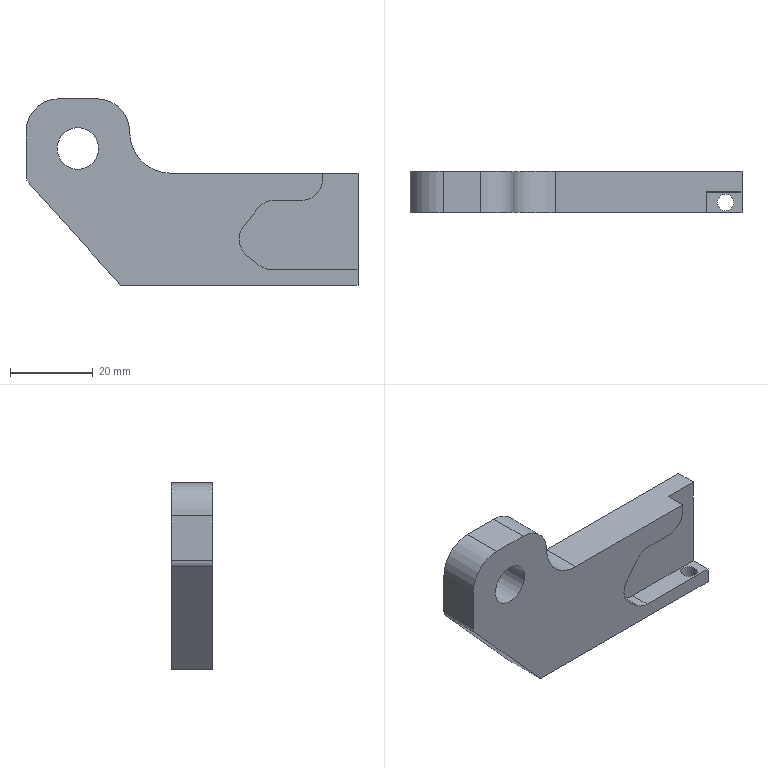Component | NX | MODEL4 | 1 solid | 24 faces | volume 19824 mm3 | plane 14 | cylinder 10 | commonest cylinder face diameters 10 x5 4 x2 16 x2 20 x1